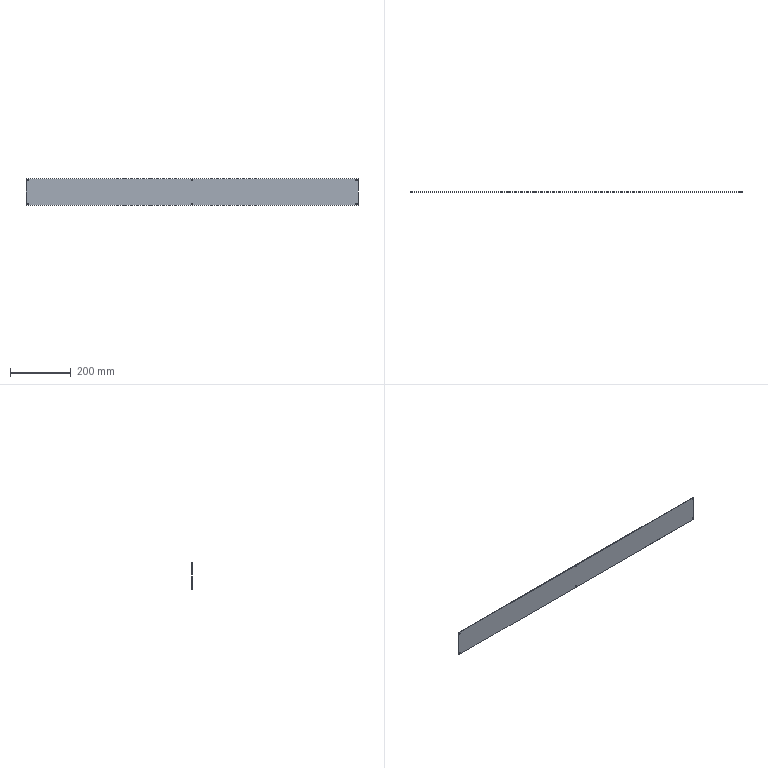Component | SolidWorks | ElectricalBoxCoverPlate-1 | 1 solid | 18 faces | box 1089 x 2 x 88 mm | volume 191513 mm3 | cylinder 12 | plane 6 | commonest cylinder face diameters 4 x12
build123d program:
from build123d import *

# Parameters (mm, degrees)
SKETCH1_W           = 1089
SKETCH1_H           = 88
BOSS_EXTRUDE1_DEPTH = 2
SKETCH2_R           = 2
CUT_EXTRUDE1_DEPTH  = 10
LPATTERN1_COUNT     = 3
LPATTERN1_PITCH     = 539.5


with BuildPart() as part:
    # Sketch1 → Boss-Extrude1 (new body)
    with BuildSketch(Plane.XY):
        with Locations((478.828, -17.742)):
            Rectangle(SKETCH1_W, SKETCH1_H)
    extrude(amount=BOSS_EXTRUDE1_DEPTH)

    # Sketch2 → Cut-Extrude1 (cut)
    with BuildSketch(Plane.XY.offset(2)):
        with Locations((-60.672, 21.258)):
            Circle(SKETCH2_R)
        with Locations((-60.672, -56.742)):
            Circle(SKETCH2_R)
    cut_extrude1 = extrude(amount=-CUT_EXTRUDE1_DEPTH, mode=Mode.SUBTRACT)

    # LPattern1: Cut-Extrude1 ×3
    with Locations(*[(i * LPATTERN1_PITCH, 0, 0) for i in range(1, LPATTERN1_COUNT)]):
        add(cut_extrude1, mode=Mode.SUBTRACT)


solid = part.part

# Placed as in the assembly
solid = solid.moved(Location((-747.877, 541.566, -160.777), (90, 0, 0)))
STEP:
#1=CARTESIAN_POINT('',(10.569,21.243,-5.493));
#2=VERTEX_POINT('',#1);
#3=CARTESIAN_POINT('',(10.726,21.243,-5.493));
#4=VERTEX_POINT('',#3);
#5=CARTESIAN_POINT('',(10.648,21.243,-5.493));
#6=DIRECTION('',(0.,1.,0.));
#7=DIRECTION('',(1.,0.,0.));
#8=AXIS2_PLACEMENT_3D('',#5,#6,#7);
#9=CIRCLE('',#8,0.07874);
#10=EDGE_CURVE('',#2,#4,#9,.T.);
#11=ORIENTED_EDGE('',*,*,#10,.F.);
#12=CARTESIAN_POINT('',(10.569,21.322,-5.493));
#13=VERTEX_POINT('',#12);
#14=CARTESIAN_POINT('',(10.569,20.928,-5.493));
#15=DIRECTION('',(0.,1.,0.));
#16=VECTOR('',#15,39.37);
#17=LINE('',#14,#16);
#18=EDGE_CURVE('',#2,#13,#17,.T.);
#19=ORIENTED_EDGE('',*,*,#18,.T.);
#20=CARTESIAN_POINT('',(10.726,21.322,-5.493));
#21=VERTEX_POINT('',#20);
#22=CARTESIAN_POINT('',(10.648,21.322,-5.493));
#23=DIRECTION('',(0.,1.,0.));
#24=DIRECTION('',(1.,0.,0.));
#25=AXIS2_PLACEMENT_3D('',#22,#23,#24);
#26=CIRCLE('',#25,0.07874);
#27=EDGE_CURVE('',#13,#21,#26,.T.);
#28=ORIENTED_EDGE('',*,*,#27,.T.);
#29=CARTESIAN_POINT('',(10.726,20.928,-5.493));
#30=DIRECTION('',(0.,1.,0.));
#31=VECTOR('',#30,39.37);
#32=LINE('',#29,#31);
#33=EDGE_CURVE('',#4,#21,#32,.T.);
#34=ORIENTED_EDGE('',*,*,#33,.F.);
#35=EDGE_LOOP('',(#11,#19,#28,#34));
#36=FACE_OUTER_BOUND('',#35,.T.);
#37=CARTESIAN_POINT('',(10.648,20.928,-5.493));
#38=DIRECTION('',(0.,1.,0.));
#39=DIRECTION('',(1.,0.,0.));
#40=AXIS2_PLACEMENT_3D('',#37,#38,#39);
#41=CYLINDRICAL_SURFACE('',#40,0.07874);
#42=ADVANCED_FACE('',(#36),#41,.F.);
#43=CARTESIAN_POINT('',(10.569,21.243,-8.564));
#44=VERTEX_POINT('',#43);
#45=CARTESIAN_POINT('',(10.726,21.243,-8.564));
#46=VERTEX_POINT('',#45);
#47=CARTESIAN_POINT('',(10.648,21.243,-8.564));
#48=DIRECTION('',(0.,1.,0.));
#49=DIRECTION('',(1.,0.,0.));
#50=AXIS2_PLACEMENT_3D('',#47,#48,#49);
#51=CIRCLE('',#50,0.07874);
#52=EDGE_CURVE('',#44,#46,#51,.T.);
#53=ORIENTED_EDGE('',*,*,#52,.F.);
#54=CARTESIAN_POINT('',(10.569,21.322,-8.564));
#55=VERTEX_POINT('',#54);
#56=CARTESIAN_POINT('',(10.569,20.928,-8.564));
#57=DIRECTION('',(0.,1.,0.));
#58=VECTOR('',#57,39.37);
#59=LINE('',#56,#58);
#60=EDGE_CURVE('',#44,#55,#59,.T.);
#61=ORIENTED_EDGE('',*,*,#60,.T.);
#62=CARTESIAN_POINT('',(10.726,21.322,-8.564));
#63=VERTEX_POINT('',#62);
#64=CARTESIAN_POINT('',(10.648,21.322,-8.564));
#65=DIRECTION('',(0.,1.,0.));
#66=DIRECTION('',(1.,0.,0.));
#67=AXIS2_PLACEMENT_3D('',#64,#65,#66);
#68=CIRCLE('',#67,0.07874);
#69=EDGE_CURVE('',#55,#63,#68,.T.);
#70=ORIENTED_EDGE('',*,*,#69,.T.);
#71=CARTESIAN_POINT('',(10.726,20.928,-8.564));
#72=DIRECTION('',(0.,1.,0.));
#73=VECTOR('',#72,39.37);
#74=LINE('',#71,#73);
#75=EDGE_CURVE('',#46,#63,#74,.T.);
#76=ORIENTED_EDGE('',*,*,#75,.F.);
#77=EDGE_LOOP('',(#53,#61,#70,#76));
#78=FACE_OUTER_BOUND('',#77,.T.);
#79=CARTESIAN_POINT('',(10.648,20.928,-8.564));
#80=DIRECTION('',(0.,1.,0.));
#81=DIRECTION('',(1.,0.,0.));
#82=AXIS2_PLACEMENT_3D('',#79,#80,#81);
#83=CYLINDRICAL_SURFACE('',#82,0.07874);
#84=ADVANCED_FACE('',(#78),#83,.F.);
#85=CARTESIAN_POINT('',(-10.671,21.243,-5.493));
#86=VERTEX_POINT('',#85);
#87=CARTESIAN_POINT('',(-10.514,21.243,-5.493));
#88=VERTEX_POINT('',#87);
#89=CARTESIAN_POINT('',(-10.593,21.243,-5.493));
#90=DIRECTION('',(0.,1.,0.));
#91=DIRECTION('',(1.,0.,0.));
#92=AXIS2_PLACEMENT_3D('',#89,#90,#91);
#93=CIRCLE('',#92,0.07874);
#94=EDGE_CURVE('',#86,#88,#93,.T.);
#95=ORIENTED_EDGE('',*,*,#94,.F.);
#96=CARTESIAN_POINT('',(-10.671,21.322,-5.493));
#97=VERTEX_POINT('',#96);
#98=CARTESIAN_POINT('',(-10.671,20.928,-5.493));
#99=DIRECTION('',(0.,1.,0.));
#100=VECTOR('',#99,39.37);
#101=LINE('',#98,#100);
#102=EDGE_CURVE('',#86,#97,#101,.T.);
#103=ORIENTED_EDGE('',*,*,#102,.T.);
#104=CARTESIAN_POINT('',(-10.514,21.322,-5.493));
#105=VERTEX_POINT('',#104);
#106=CARTESIAN_POINT('',(-10.593,21.322,-5.493));
#107=DIRECTION('',(0.,1.,0.));
#108=DIRECTION('',(1.,0.,0.));
#109=AXIS2_PLACEMENT_3D('',#106,#107,#108);
#110=CIRCLE('',#109,0.07874);
#111=EDGE_CURVE('',#97,#105,#110,.T.);
#112=ORIENTED_EDGE('',*,*,#111,.T.);
#113=CARTESIAN_POINT('',(-10.514,20.928,-5.493));
#114=DIRECTION('',(0.,1.,0.));
#115=VECTOR('',#114,39.37);
#116=LINE('',#113,#115);
#117=EDGE_CURVE('',#88,#105,#116,.T.);
#118=ORIENTED_EDGE('',*,*,#117,.F.);
#119=EDGE_LOOP('',(#95,#103,#112,#118));
#120=FACE_OUTER_BOUND('',#119,.T.);
#121=CARTESIAN_POINT('',(-10.593,20.928,-5.493));
#122=DIRECTION('',(0.,1.,0.));
#123=DIRECTION('',(1.,0.,0.));
#124=AXIS2_PLACEMENT_3D('',#121,#122,#123);
#125=CYLINDRICAL_SURFACE('',#124,0.07874);
#126=ADVANCED_FACE('',(#120),#125,.F.);
#127=CARTESIAN_POINT('',(-10.671,21.243,-8.564));
#128=VERTEX_POINT('',#127);
#129=CARTESIAN_POINT('',(-10.514,21.243,-8.564));
#130=VERTEX_POINT('',#129);
#131=CARTESIAN_POINT('',(-10.593,21.243,-8.564));
#132=DIRECTION('',(0.,1.,0.));
#133=DIRECTION('',(1.,0.,0.));
#134=AXIS2_PLACEMENT_3D('',#131,#132,#133);
#135=CIRCLE('',#134,0.07874);
#136=EDGE_CURVE('',#128,#130,#135,.T.);
#137=ORIENTED_EDGE('',*,*,#136,.F.);
#138=CARTESIAN_POINT('',(-10.671,21.322,-8.564));
#139=VERTEX_POINT('',#138);
#140=CARTESIAN_POINT('',(-10.671,20.928,-8.564));
#141=DIRECTION('',(0.,1.,0.));
#142=VECTOR('',#141,39.37);
#143=LINE('',#140,#142);
#144=EDGE_CURVE('',#128,#139,#143,.T.);
#145=ORIENTED_EDGE('',*,*,#144,.T.);
#146=CARTESIAN_POINT('',(-10.514,21.322,-8.564));
#147=VERTEX_POINT('',#146);
#148=CARTESIAN_POINT('',(-10.593,21.322,-8.564));
#149=DIRECTION('',(0.,1.,0.));
#150=DIRECTION('',(1.,0.,0.));
#151=AXIS2_PLACEMENT_3D('',#148,#149,#150);
#152=CIRCLE('',#151,0.07874);
#153=EDGE_CURVE('',#139,#147,#152,.T.);
#154=ORIENTED_EDGE('',*,*,#153,.T.);
#155=CARTESIAN_POINT('',(-10.514,20.928,-8.564));
#156=DIRECTION('',(0.,1.,0.));
#157=VECTOR('',#156,39.37);
#158=LINE('',#155,#157);
#159=EDGE_CURVE('',#130,#147,#158,.T.);
#160=ORIENTED_EDGE('',*,*,#159,.F.);
#161=EDGE_LOOP('',(#137,#145,#154,#160));
#162=FACE_OUTER_BOUND('',#161,.T.);
#163=CARTESIAN_POINT('',(-10.593,20.928,-8.564));
#164=DIRECTION('',(0.,1.,0.));
#165=DIRECTION('',(1.,0.,0.));
#166=AXIS2_PLACEMENT_3D('',#163,#164,#165);
#167=CYLINDRICAL_SURFACE('',#166,0.07874);
#168=ADVANCED_FACE('',(#162),#167,.F.);
#169=CARTESIAN_POINT('',(-31.911,21.243,-5.493));
#170=VERTEX_POINT('',#169);
#171=CARTESIAN_POINT('',(-31.754,21.243,-5.493));
#172=VERTEX_POINT('',#171);
#173=CARTESIAN_POINT('',(-31.833,21.243,-5.493));
#174=DIRECTION('',(0.,1.,0.));
#175=DIRECTION('',(1.,0.,0.));
#176=AXIS2_PLACEMENT_3D('',#173,#174,#175);
#177=CIRCLE('',#176,0.07874);
#178=EDGE_CURVE('',#170,#172,#177,.T.);
#179=ORIENTED_EDGE('',*,*,#178,.F.);
#180=CARTESIAN_POINT('',(-31.911,21.322,-5.493));
#181=VERTEX_POINT('',#180);
#182=CARTESIAN_POINT('',(-31.911,20.928,-5.493));
#183=DIRECTION('',(0.,1.,0.));
#184=VECTOR('',#183,39.37);
#185=LINE('',#182,#184);
#186=EDGE_CURVE('',#170,#181,#185,.T.);
#187=ORIENTED_EDGE('',*,*,#186,.T.);
#188=CARTESIAN_POINT('',(-31.754,21.322,-5.493));
#189=VERTEX_POINT('',#188);
#190=CARTESIAN_POINT('',(-31.833,21.322,-5.493));
#191=DIRECTION('',(0.,1.,0.));
#192=DIRECTION('',(1.,0.,0.));
#193=AXIS2_PLACEMENT_3D('',#190,#191,#192);
#194=CIRCLE('',#193,0.07874);
#195=EDGE_CURVE('',#181,#189,#194,.T.);
#196=ORIENTED_EDGE('',*,*,#195,.T.);
#197=CARTESIAN_POINT('',(-31.754,20.928,-5.493));
#198=DIRECTION('',(0.,1.,0.));
#199=VECTOR('',#198,39.37);
#200=LINE('',#197,#199);
#201=EDGE_CURVE('',#172,#189,#200,.T.);
#202=ORIENTED_EDGE('',*,*,#201,.F.);
#203=EDGE_LOOP('',(#179,#187,#196,#202));
#204=FACE_OUTER_BOUND('',#203,.T.);
#205=CARTESIAN_POINT('',(-31.833,20.928,-5.493));
#206=DIRECTION('',(0.,1.,0.));
#207=DIRECTION('',(1.,0.,0.));
#208=AXIS2_PLACEMENT_3D('',#205,#206,#207);
#209=CYLINDRICAL_SURFACE('',#208,0.07874);
#210=ADVANCED_FACE('',(#204),#209,.F.);
#211=CARTESIAN_POINT('',(-31.911,21.243,-8.564));
#212=VERTEX_POINT('',#211);
#213=CARTESIAN_POINT('',(-31.754,21.243,-8.564));
#214=VERTEX_POINT('',#213);
#215=CARTESIAN_POINT('',(-31.833,21.243,-8.564));
#216=DIRECTION('',(0.,1.,0.));
#217=DIRECTION('',(1.,0.,0.));
#218=AXIS2_PLACEMENT_3D('',#215,#216,#217);
#219=CIRCLE('',#218,0.07874);
#220=EDGE_CURVE('',#212,#214,#219,.T.);
#221=ORIENTED_EDGE('',*,*,#220,.F.);
#222=CARTESIAN_POINT('',(-31.911,21.322,-8.564));
#223=VERTEX_POINT('',#222);
#224=CARTESIAN_POINT('',(-31.911,20.928,-8.564));
#225=DIRECTION('',(0.,1.,0.));
#226=VECTOR('',#225,39.37);
#227=LINE('',#224,#226);
#228=EDGE_CURVE('',#212,#223,#227,.T.);
#229=ORIENTED_EDGE('',*,*,#228,.T.);
#230=CARTESIAN_POINT('',(-31.754,21.322,-8.564));
#231=VERTEX_POINT('',#230);
#232=CARTESIAN_POINT('',(-31.833,21.322,-8.564));
#233=DIRECTION('',(0.,1.,0.));
#234=DIRECTION('',(1.,0.,0.));
#235=AXIS2_PLACEMENT_3D('',#232,#233,#234);
#236=CIRCLE('',#235,0.07874);
#237=EDGE_CURVE('',#223,#231,#236,.T.);
#238=ORIENTED_EDGE('',*,*,#237,.T.);
#239=CARTESIAN_POINT('',(-31.754,20.928,-8.564));
#240=DIRECTION('',(0.,1.,0.));
#241=VECTOR('',#240,39.37);
#242=LINE('',#239,#241);
#243=EDGE_CURVE('',#214,#231,#242,.T.);
#244=ORIENTED_EDGE('',*,*,#243,.F.);
#245=EDGE_LOOP('',(#221,#229,#238,#244));
#246=FACE_OUTER_BOUND('',#245,.T.);
#247=CARTESIAN_POINT('',(-31.833,20.928,-8.564));
#248=DIRECTION('',(0.,1.,0.));
#249=DIRECTION('',(1.,0.,0.));
#250=AXIS2_PLACEMENT_3D('',#247,#248,#249);
#251=CYLINDRICAL_SURFACE('',#250,0.07874);
#252=ADVANCED_FACE('',(#246),#251,.F.);
#253=CARTESIAN_POINT('',(-32.03,21.243,-8.761));
#254=VERTEX_POINT('',#253);
#255=CARTESIAN_POINT('',(-32.03,21.243,-5.296));
#256=VERTEX_POINT('',#255);
#257=CARTESIAN_POINT('',(-32.03,21.243,-8.761));
#258=DIRECTION('',(0.,-0.,1.));
#259=VECTOR('',#258,39.37);
#260=LINE('',#257,#259);
#261=EDGE_CURVE('',#254,#256,#260,.T.);
#262=ORIENTED_EDGE('',*,*,#261,.T.);
#263=CARTESIAN_POINT('',(-32.03,21.322,-5.296));
#264=VERTEX_POINT('',#263);
#265=CARTESIAN_POINT('',(-32.03,21.322,-5.296));
#266=DIRECTION('',(-0.,-1.,-0.));
#267=VECTOR('',#266,39.37);
#268=LINE('',#265,#267);
#269=EDGE_CURVE('',#264,#256,#268,.T.);
#270=ORIENTED_EDGE('',*,*,#269,.F.);
#271=CARTESIAN_POINT('',(-32.03,21.322,-8.761));
#272=VERTEX_POINT('',#271);
#273=CARTESIAN_POINT('',(-32.03,21.322,-8.761));
#274=DIRECTION('',(0.,-0.,1.));
#275=VECTOR('',#274,39.37);
#276=LINE('',#273,#275);
#277=EDGE_CURVE('',#272,#264,#276,.T.);
#278=ORIENTED_EDGE('',*,*,#277,.F.);
#279=CARTESIAN_POINT('',(-32.03,21.322,-8.761));
#280=DIRECTION('',(-0.,-1.,-0.));
#281=VECTOR('',#280,39.37);
#282=LINE('',#279,#281);
#283=EDGE_CURVE('',#272,#254,#282,.T.);
#284=ORIENTED_EDGE('',*,*,#283,.T.);
#285=EDGE_LOOP('',(#262,#270,#278,#284));
#286=FACE_OUTER_BOUND('',#285,.T.);
#287=CARTESIAN_POINT('',(-32.03,21.322,-8.761));
#288=DIRECTION('',(1.,0.,-0.));
#289=DIRECTION('',(-0.,0.,-1.));
#290=AXIS2_PLACEMENT_3D('',#287,#288,#289);
#291=PLANE('',#290);
#292=ADVANCED_FACE('',(#286),#291,.F.);
#293=CARTESIAN_POINT('',(10.845,21.243,-5.296));
#294=VERTEX_POINT('',#293);
#295=CARTESIAN_POINT('',(-32.03,21.243,-5.296));
#296=DIRECTION('',(1.,0.,0.));
#297=VECTOR('',#296,39.37);
#298=LINE('',#295,#297);
#299=EDGE_CURVE('',#256,#294,#298,.T.);
#300=ORIENTED_EDGE('',*,*,#299,.T.);
#301=CARTESIAN_POINT('',(10.845,21.322,-5.296));
#302=VERTEX_POINT('',#301);
#303=CARTESIAN_POINT('',(10.845,21.322,-5.296));
#304=DIRECTION('',(-0.,-1.,-0.));
#305=VECTOR('',#304,39.37);
#306=LINE('',#303,#305);
#307=EDGE_CURVE('',#302,#294,#306,.T.);
#308=ORIENTED_EDGE('',*,*,#307,.F.);
#309=CARTESIAN_POINT('',(-32.03,21.322,-5.296));
#310=DIRECTION('',(1.,0.,0.));
#311=VECTOR('',#310,39.37);
#312=LINE('',#309,#311);
#313=EDGE_CURVE('',#264,#302,#312,.T.);
#314=ORIENTED_EDGE('',*,*,#313,.F.);
#315=ORIENTED_EDGE('',*,*,#269,.T.);
#316=EDGE_LOOP('',(#300,#308,#314,#315));
#317=FACE_OUTER_BOUND('',#316,.T.);
#318=CARTESIAN_POINT('',(-32.03,21.322,-5.296));
#319=DIRECTION('',(0.,0.,-1.));
#320=DIRECTION('',(0.,1.,0.));
#321=AXIS2_PLACEMENT_3D('',#318,#319,#320);
#322=PLANE('',#321);
#323=ADVANCED_FACE('',(#317),#322,.F.);
#324=CARTESIAN_POINT('',(10.845,21.243,-8.761));
#325=VERTEX_POINT('',#324);
#326=CARTESIAN_POINT('',(10.845,21.243,-8.761));
#327=DIRECTION('',(0.,0.,-1.));
#328=VECTOR('',#327,39.37);
#329=LINE('',#326,#328);
#330=EDGE_CURVE('',#294,#325,#329,.T.);
#331=ORIENTED_EDGE('',*,*,#330,.T.);
#332=CARTESIAN_POINT('',(10.845,21.322,-8.761));
#333=VERTEX_POINT('',#332);
#334=CARTESIAN_POINT('',(10.845,21.322,-8.761));
#335=DIRECTION('',(-0.,-1.,-0.));
#336=VECTOR('',#335,39.37);
#337=LINE('',#334,#336);
#338=EDGE_CURVE('',#333,#325,#337,.T.);
#339=ORIENTED_EDGE('',*,*,#338,.F.);
#340=CARTESIAN_POINT('',(10.845,21.322,-8.761));
#341=DIRECTION('',(0.,0.,-1.));
#342=VECTOR('',#341,39.37);
#343=LINE('',#340,#342);
#344=EDGE_CURVE('',#302,#333,#343,.T.);
#345=ORIENTED_EDGE('',*,*,#344,.F.);
#346=ORIENTED_EDGE('',*,*,#307,.T.);
#347=EDGE_LOOP('',(#331,#339,#345,#346));
#348=FACE_OUTER_BOUND('',#347,.T.);
#349=CARTESIAN_POINT('',(10.845,21.322,-8.761));
#350=DIRECTION('',(-1.,0.,0.));
#351=DIRECTION('',(0.,1.,0.));
#352=AXIS2_PLACEMENT_3D('',#349,#350,#351);
#353=PLANE('',#352);
#354=ADVANCED_FACE('',(#348),#353,.F.);
#355=CARTESIAN_POINT('',(-32.03,21.243,-8.761));
#356=DIRECTION('',(-1.,0.,0.));
#357=VECTOR('',#356,39.37);
#358=LINE('',#355,#357);
#359=EDGE_CURVE('',#325,#254,#358,.T.);
#360=ORIENTED_EDGE('',*,*,#359,.T.);
#361=ORIENTED_EDGE('',*,*,#283,.F.);
#362=CARTESIAN_POINT('',(-32.03,21.322,-8.761));
#363=DIRECTION('',(-1.,0.,0.));
#364=VECTOR('',#363,39.37);
#365=LINE('',#362,#364);
#366=EDGE_CURVE('',#333,#272,#365,.T.);
#367=ORIENTED_EDGE('',*,*,#366,.F.);
#368=ORIENTED_EDGE('',*,*,#338,.T.);
#369=EDGE_LOOP('',(#360,#361,#367,#368));
#370=FACE_OUTER_BOUND('',#369,.T.);
#371=CARTESIAN_POINT('',(-32.03,21.322,-8.761));
#372=DIRECTION('',(-0.,-0.,1.));
#373=DIRECTION('',(-0.,-1.,-0.));
#374=AXIS2_PLACEMENT_3D('',#371,#372,#373);
#375=PLANE('',#374);
#376=ADVANCED_FACE('',(#370),#375,.F.);
#377=CARTESIAN_POINT('',(-10.593,21.322,-5.493));
#378=DIRECTION('',(0.,1.,0.));
#379=DIRECTION('',(1.,0.,0.));
#380=AXIS2_PLACEMENT_3D('',#377,#378,#379);
#381=CIRCLE('',#380,0.07874);
#382=EDGE_CURVE('',#105,#97,#381,.T.);
#383=ORIENTED_EDGE('',*,*,#382,.F.);
#384=ORIENTED_EDGE('',*,*,#111,.F.);
#385=EDGE_LOOP('',(#383,#384));
#386=FACE_BOUND('',#385,.T.);
#387=CARTESIAN_POINT('',(-10.593,21.322,-8.564));
#388=DIRECTION('',(0.,1.,0.));
#389=DIRECTION('',(1.,0.,0.));
#390=AXIS2_PLACEMENT_3D('',#387,#388,#389);
#391=CIRCLE('',#390,0.07874);
#392=EDGE_CURVE('',#147,#139,#391,.T.);
#393=ORIENTED_EDGE('',*,*,#392,.F.);
#394=ORIENTED_EDGE('',*,*,#153,.F.);
#395=EDGE_LOOP('',(#393,#394));
#396=FACE_BOUND('',#395,.T.);
#397=CARTESIAN_POINT('',(-31.833,21.322,-5.493));
#398=DIRECTION('',(0.,1.,0.));
#399=DIRECTION('',(1.,0.,0.));
#400=AXIS2_PLACEMENT_3D('',#397,#398,#399);
#401=CIRCLE('',#400,0.07874);
#402=EDGE_CURVE('',#189,#181,#401,.T.);
#403=ORIENTED_EDGE('',*,*,#402,.F.);
#404=ORIENTED_EDGE('',*,*,#195,.F.);
#405=EDGE_LOOP('',(#403,#404));
#406=FACE_BOUND('',#405,.T.);
#407=CARTESIAN_POINT('',(-31.833,21.322,-8.564));
#408=DIRECTION('',(0.,1.,0.));
#409=DIRECTION('',(1.,0.,0.));
#410=AXIS2_PLACEMENT_3D('',#407,#408,#409);
#411=CIRCLE('',#410,0.07874);
#412=EDGE_CURVE('',#231,#223,#411,.T.);
#413=ORIENTED_EDGE('',*,*,#412,.F.);
#414=ORIENTED_EDGE('',*,*,#237,.F.);
#415=EDGE_LOOP('',(#413,#414));
#416=FACE_BOUND('',#415,.T.);
#417=ORIENTED_EDGE('',*,*,#277,.T.);
#418=ORIENTED_EDGE('',*,*,#313,.T.);
#419=ORIENTED_EDGE('',*,*,#344,.T.);
#420=ORIENTED_EDGE('',*,*,#366,.T.);
#421=EDGE_LOOP('',(#417,#418,#419,#420));
#422=FACE_OUTER_BOUND('',#421,.T.);
#423=CARTESIAN_POINT('',(10.648,21.322,-8.564));
#424=DIRECTION('',(0.,1.,0.));
#425=DIRECTION('',(1.,0.,0.));
#426=AXIS2_PLACEMENT_3D('',#423,#424,#425);
#427=CIRCLE('',#426,0.07874);
#428=EDGE_CURVE('',#63,#55,#427,.T.);
#429=ORIENTED_EDGE('',*,*,#428,.F.);
#430=ORIENTED_EDGE('',*,*,#69,.F.);
#431=EDGE_LOOP('',(#429,#430));
#432=FACE_BOUND('',#431,.T.);
#433=CARTESIAN_POINT('',(10.648,21.322,-5.493));
#434=DIRECTION('',(0.,1.,0.));
#435=DIRECTION('',(1.,0.,0.));
#436=AXIS2_PLACEMENT_3D('',#433,#434,#435);
#437=CIRCLE('',#436,0.07874);
#438=EDGE_CURVE('',#21,#13,#437,.T.);
#439=ORIENTED_EDGE('',*,*,#438,.F.);
#440=ORIENTED_EDGE('',*,*,#27,.F.);
#441=EDGE_LOOP('',(#439,#440));
#442=FACE_BOUND('',#441,.T.);
#443=CARTESIAN_POINT('',(-29.444,21.322,-7.727));
#444=DIRECTION('',(0.,1.,0.));
#445=DIRECTION('',(1.,0.,0.));
#446=AXIS2_PLACEMENT_3D('',#443,#444,#445);
#447=PLANE('',#446);
#448=ADVANCED_FACE('',(#386,#396,#406,#416,#422,#432,#442),#447,.T.);
#449=CARTESIAN_POINT('',(-10.593,21.243,-5.493));
#450=DIRECTION('',(0.,1.,0.));
#451=DIRECTION('',(1.,0.,0.));
#452=AXIS2_PLACEMENT_3D('',#449,#450,#451);
#453=CIRCLE('',#452,0.07874);
#454=EDGE_CURVE('',#88,#86,#453,.T.);
#455=ORIENTED_EDGE('',*,*,#454,.T.);
#456=ORIENTED_EDGE('',*,*,#94,.T.);
#457=EDGE_LOOP('',(#455,#456));
#458=FACE_BOUND('',#457,.T.);
#459=CARTESIAN_POINT('',(-10.593,21.243,-8.564));
#460=DIRECTION('',(0.,1.,0.));
#461=DIRECTION('',(1.,0.,0.));
#462=AXIS2_PLACEMENT_3D('',#459,#460,#461);
#463=CIRCLE('',#462,0.07874);
#464=EDGE_CURVE('',#130,#128,#463,.T.);
#465=ORIENTED_EDGE('',*,*,#464,.T.);
#466=ORIENTED_EDGE('',*,*,#136,.T.);
#467=EDGE_LOOP('',(#465,#466));
#468=FACE_BOUND('',#467,.T.);
#469=CARTESIAN_POINT('',(-31.833,21.243,-5.493));
#470=DIRECTION('',(0.,1.,0.));
#471=DIRECTION('',(1.,0.,0.));
#472=AXIS2_PLACEMENT_3D('',#469,#470,#471);
#473=CIRCLE('',#472,0.07874);
#474=EDGE_CURVE('',#172,#170,#473,.T.);
#475=ORIENTED_EDGE('',*,*,#474,.T.);
#476=ORIENTED_EDGE('',*,*,#178,.T.);
#477=EDGE_LOOP('',(#475,#476));
#478=FACE_BOUND('',#477,.T.);
#479=CARTESIAN_POINT('',(-31.833,21.243,-8.564));
#480=DIRECTION('',(0.,1.,0.));
#481=DIRECTION('',(1.,0.,0.));
#482=AXIS2_PLACEMENT_3D('',#479,#480,#481);
#483=CIRCLE('',#482,0.07874);
#484=EDGE_CURVE('',#214,#212,#483,.T.);
#485=ORIENTED_EDGE('',*,*,#484,.T.);
#486=ORIENTED_EDGE('',*,*,#220,.T.);
#487=EDGE_LOOP('',(#485,#486));
#488=FACE_BOUND('',#487,.T.);
#489=ORIENTED_EDGE('',*,*,#261,.F.);
#490=ORIENTED_EDGE('',*,*,#359,.F.);
#491=ORIENTED_EDGE('',*,*,#330,.F.);
#492=ORIENTED_EDGE('',*,*,#299,.F.);
#493=EDGE_LOOP('',(#489,#490,#491,#492));
#494=FACE_OUTER_BOUND('',#493,.T.);
#495=CARTESIAN_POINT('',(10.648,21.243,-8.564));
#496=DIRECTION('',(0.,1.,0.));
#497=DIRECTION('',(1.,0.,0.));
#498=AXIS2_PLACEMENT_3D('',#495,#496,#497);
#499=CIRCLE('',#498,0.07874);
#500=EDGE_CURVE('',#46,#44,#499,.T.);
#501=ORIENTED_EDGE('',*,*,#500,.T.);
#502=ORIENTED_EDGE('',*,*,#52,.T.);
#503=EDGE_LOOP('',(#501,#502));
#504=FACE_BOUND('',#503,.T.);
#505=CARTESIAN_POINT('',(10.648,21.243,-5.493));
#506=DIRECTION('',(0.,1.,0.));
#507=DIRECTION('',(1.,0.,0.));
#508=AXIS2_PLACEMENT_3D('',#505,#506,#507);
#509=CIRCLE('',#508,0.07874);
#510=EDGE_CURVE('',#4,#2,#509,.T.);
#511=ORIENTED_EDGE('',*,*,#510,.T.);
#512=ORIENTED_EDGE('',*,*,#10,.T.);
#513=EDGE_LOOP('',(#511,#512));
#514=FACE_BOUND('',#513,.T.);
#515=CARTESIAN_POINT('',(-29.444,21.243,-7.727));
#516=DIRECTION('',(0.,1.,0.));
#517=DIRECTION('',(1.,0.,0.));
#518=AXIS2_PLACEMENT_3D('',#515,#516,#517);
#519=PLANE('',#518);
#520=ADVANCED_FACE('',(#458,#468,#478,#488,#494,#504,#514),#519,.F.);
#521=ORIENTED_EDGE('',*,*,#228,.F.);
#522=ORIENTED_EDGE('',*,*,#484,.F.);
#523=ORIENTED_EDGE('',*,*,#243,.T.);
#524=ORIENTED_EDGE('',*,*,#412,.T.);
#525=EDGE_LOOP('',(#521,#522,#523,#524));
#526=FACE_OUTER_BOUND('',#525,.T.);
#527=CARTESIAN_POINT('',(-31.833,20.928,-8.564));
#528=DIRECTION('',(0.,1.,0.));
#529=DIRECTION('',(1.,0.,0.));
#530=AXIS2_PLACEMENT_3D('',#527,#528,#529);
#531=CYLINDRICAL_SURFACE('',#530,0.07874);
#532=ADVANCED_FACE('',(#526),#531,.F.);
#533=ORIENTED_EDGE('',*,*,#186,.F.);
#534=ORIENTED_EDGE('',*,*,#474,.F.);
#535=ORIENTED_EDGE('',*,*,#201,.T.);
#536=ORIENTED_EDGE('',*,*,#402,.T.);
#537=EDGE_LOOP('',(#533,#534,#535,#536));
#538=FACE_OUTER_BOUND('',#537,.T.);
#539=CARTESIAN_POINT('',(-31.833,20.928,-5.493));
#540=DIRECTION('',(0.,1.,0.));
#541=DIRECTION('',(1.,0.,0.));
#542=AXIS2_PLACEMENT_3D('',#539,#540,#541);
#543=CYLINDRICAL_SURFACE('',#542,0.07874);
#544=ADVANCED_FACE('',(#538),#543,.F.);
#545=ORIENTED_EDGE('',*,*,#144,.F.);
#546=ORIENTED_EDGE('',*,*,#464,.F.);
#547=ORIENTED_EDGE('',*,*,#159,.T.);
#548=ORIENTED_EDGE('',*,*,#392,.T.);
#549=EDGE_LOOP('',(#545,#546,#547,#548));
#550=FACE_OUTER_BOUND('',#549,.T.);
#551=CARTESIAN_POINT('',(-10.593,20.928,-8.564));
#552=DIRECTION('',(0.,1.,0.));
#553=DIRECTION('',(1.,0.,0.));
#554=AXIS2_PLACEMENT_3D('',#551,#552,#553);
#555=CYLINDRICAL_SURFACE('',#554,0.07874);
#556=ADVANCED_FACE('',(#550),#555,.F.);
#557=ORIENTED_EDGE('',*,*,#102,.F.);
#558=ORIENTED_EDGE('',*,*,#454,.F.);
#559=ORIENTED_EDGE('',*,*,#117,.T.);
#560=ORIENTED_EDGE('',*,*,#382,.T.);
#561=EDGE_LOOP('',(#557,#558,#559,#560));
#562=FACE_OUTER_BOUND('',#561,.T.);
#563=CARTESIAN_POINT('',(-10.593,20.928,-5.493));
#564=DIRECTION('',(0.,1.,0.));
#565=DIRECTION('',(1.,0.,0.));
#566=AXIS2_PLACEMENT_3D('',#563,#564,#565);
#567=CYLINDRICAL_SURFACE('',#566,0.07874);
#568=ADVANCED_FACE('',(#562),#567,.F.);
#569=ORIENTED_EDGE('',*,*,#60,.F.);
#570=ORIENTED_EDGE('',*,*,#500,.F.);
#571=ORIENTED_EDGE('',*,*,#75,.T.);
#572=ORIENTED_EDGE('',*,*,#428,.T.);
#573=EDGE_LOOP('',(#569,#570,#571,#572));
#574=FACE_OUTER_BOUND('',#573,.T.);
#575=CARTESIAN_POINT('',(10.648,20.928,-8.564));
#576=DIRECTION('',(0.,1.,0.));
#577=DIRECTION('',(1.,0.,0.));
#578=AXIS2_PLACEMENT_3D('',#575,#576,#577);
#579=CYLINDRICAL_SURFACE('',#578,0.07874);
#580=ADVANCED_FACE('',(#574),#579,.F.);
#581=ORIENTED_EDGE('',*,*,#18,.F.);
#582=ORIENTED_EDGE('',*,*,#510,.F.);
#583=ORIENTED_EDGE('',*,*,#33,.T.);
#584=ORIENTED_EDGE('',*,*,#438,.T.);
#585=EDGE_LOOP('',(#581,#582,#583,#584));
#586=FACE_OUTER_BOUND('',#585,.T.);
#587=CARTESIAN_POINT('',(10.648,20.928,-5.493));
#588=DIRECTION('',(0.,1.,0.));
#589=DIRECTION('',(1.,0.,0.));
#590=AXIS2_PLACEMENT_3D('',#587,#588,#589);
#591=CYLINDRICAL_SURFACE('',#590,0.07874);
#592=ADVANCED_FACE('',(#586),#591,.F.);
#593=CLOSED_SHELL('',(#42,#84,#126,#168,#210,#252,#292,#323,#354,#376,#448,#520,#532,#544,#556,#568,#580,#592));
#594=MANIFOLD_SOLID_BREP('',#593);
#595=CARTESIAN_POINT('',(0.,0.,0.));
#596=DIRECTION('',(0.,0.,1.));
#597=DIRECTION('',(1.,0.,0.));
#598=AXIS2_PLACEMENT_3D('',#595,#596,#597);
#599=(LENGTH_UNIT()NAMED_UNIT(*)SI_UNIT($,.METRE.));
#600=LENGTH_MEASURE_WITH_UNIT(LENGTH_MEASURE(0.0254),#599);
#601=DIMENSIONAL_EXPONENTS(1.,0.,0.,0.,0.,0.,0.);
#602=(CONVERSION_BASED_UNIT('',#600)LENGTH_UNIT()NAMED_UNIT(#601));
#603=UNCERTAINTY_MEASURE_WITH_UNIT(LENGTH_MEASURE(0.00001),#602,'','');
#604=(NAMED_UNIT(*)PLANE_ANGLE_UNIT()SI_UNIT($,.RADIAN.));
#605=(NAMED_UNIT(*)SI_UNIT($,.STERADIAN.)SOLID_ANGLE_UNIT());
#606=(GEOMETRIC_REPRESENTATION_CONTEXT(3)GLOBAL_UNCERTAINTY_ASSIGNED_CONTEXT((#603))GLOBAL_UNIT_ASSIGNED_CONTEXT((#602,#604,#605))REPRESENTATION_CONTEXT('',''));
#607=ADVANCED_BREP_SHAPE_REPRESENTATION('',(#594,#598),#606);
#608=COLOUR_RGB('',0.7922,0.8196,0.9333);
#609=FILL_AREA_STYLE_COLOUR('',#608);
#610=FILL_AREA_STYLE('',(#609));
#611=SURFACE_STYLE_FILL_AREA(#610);
#612=SURFACE_SIDE_STYLE('',(#611));
#613=SURFACE_STYLE_USAGE(.BOTH.,#612);
#614=PRESENTATION_STYLE_ASSIGNMENT((#613));
#615=STYLED_ITEM('',(#614),#594);
#616=PRESENTATION_LAYER_ASSIGNMENT('','',(#615));
#617=(LENGTH_UNIT()NAMED_UNIT(*)SI_UNIT($,.METRE.));
#618=LENGTH_MEASURE_WITH_UNIT(LENGTH_MEASURE(0.0254),#617);
#619=DIMENSIONAL_EXPONENTS(1.,0.,0.,0.,0.,0.,0.);
#620=(CONVERSION_BASED_UNIT('',#618)LENGTH_UNIT()NAMED_UNIT(#619));
#621=UNCERTAINTY_MEASURE_WITH_UNIT(LENGTH_MEASURE(0.00001),#620,'','');
#622=(NAMED_UNIT(*)PLANE_ANGLE_UNIT()SI_UNIT($,.RADIAN.));
#623=(NAMED_UNIT(*)SI_UNIT($,.STERADIAN.)SOLID_ANGLE_UNIT());
#624=(GEOMETRIC_REPRESENTATION_CONTEXT(3)GLOBAL_UNCERTAINTY_ASSIGNED_CONTEXT((#621))GLOBAL_UNIT_ASSIGNED_CONTEXT((#620,#622,#623))REPRESENTATION_CONTEXT('',''));
#625=MECHANICAL_DESIGN_GEOMETRIC_PRESENTATION_REPRESENTATION('',(#615),#624);